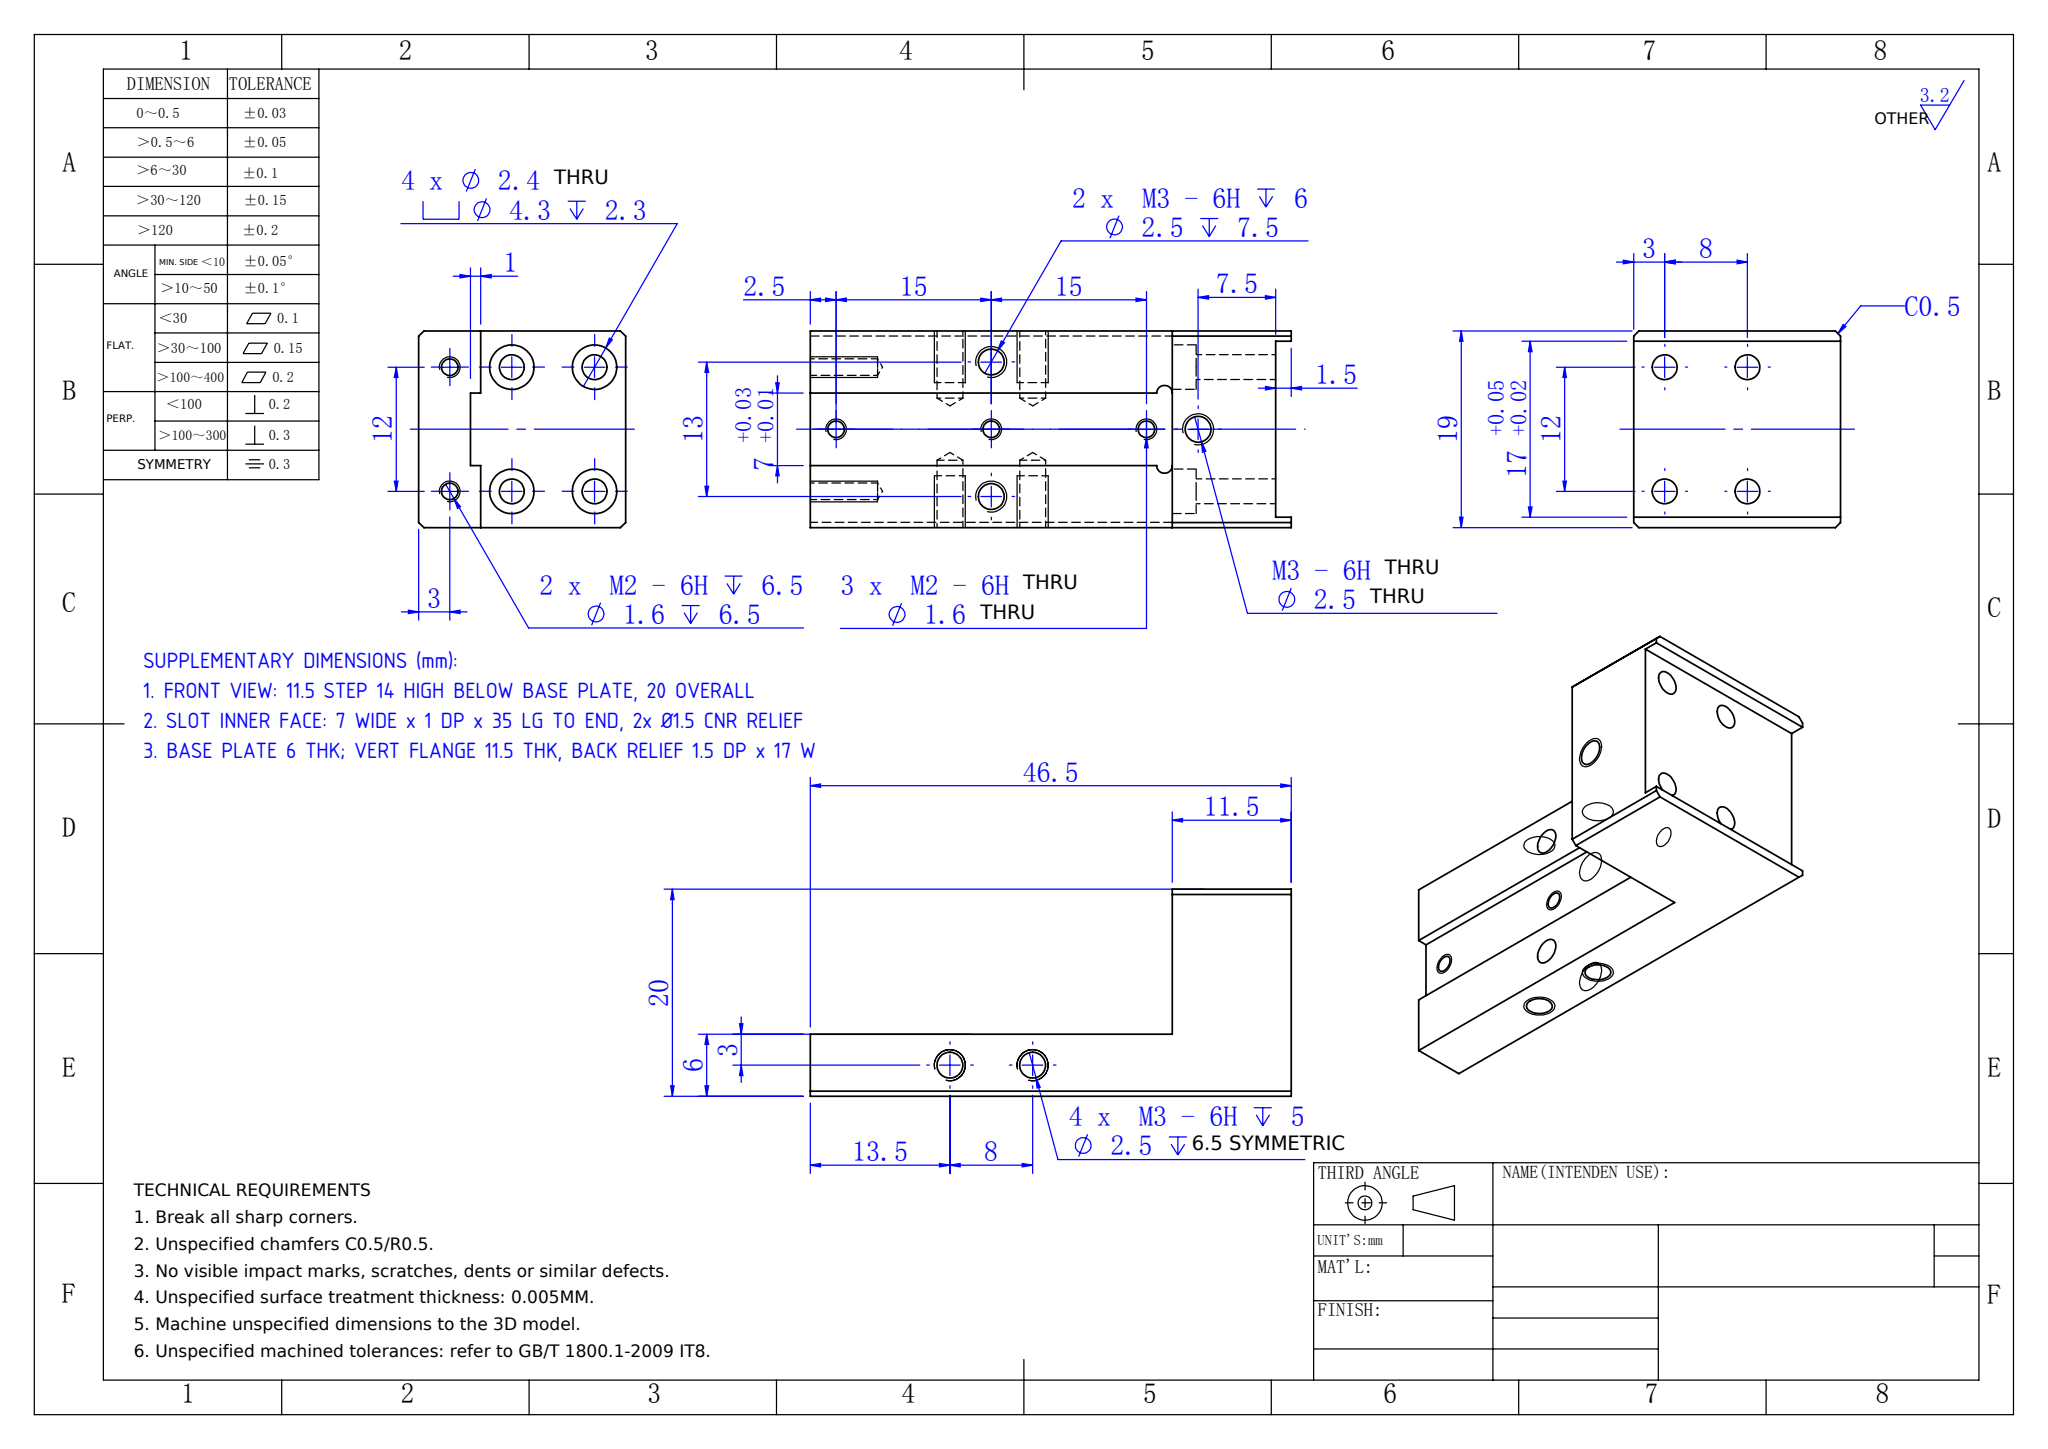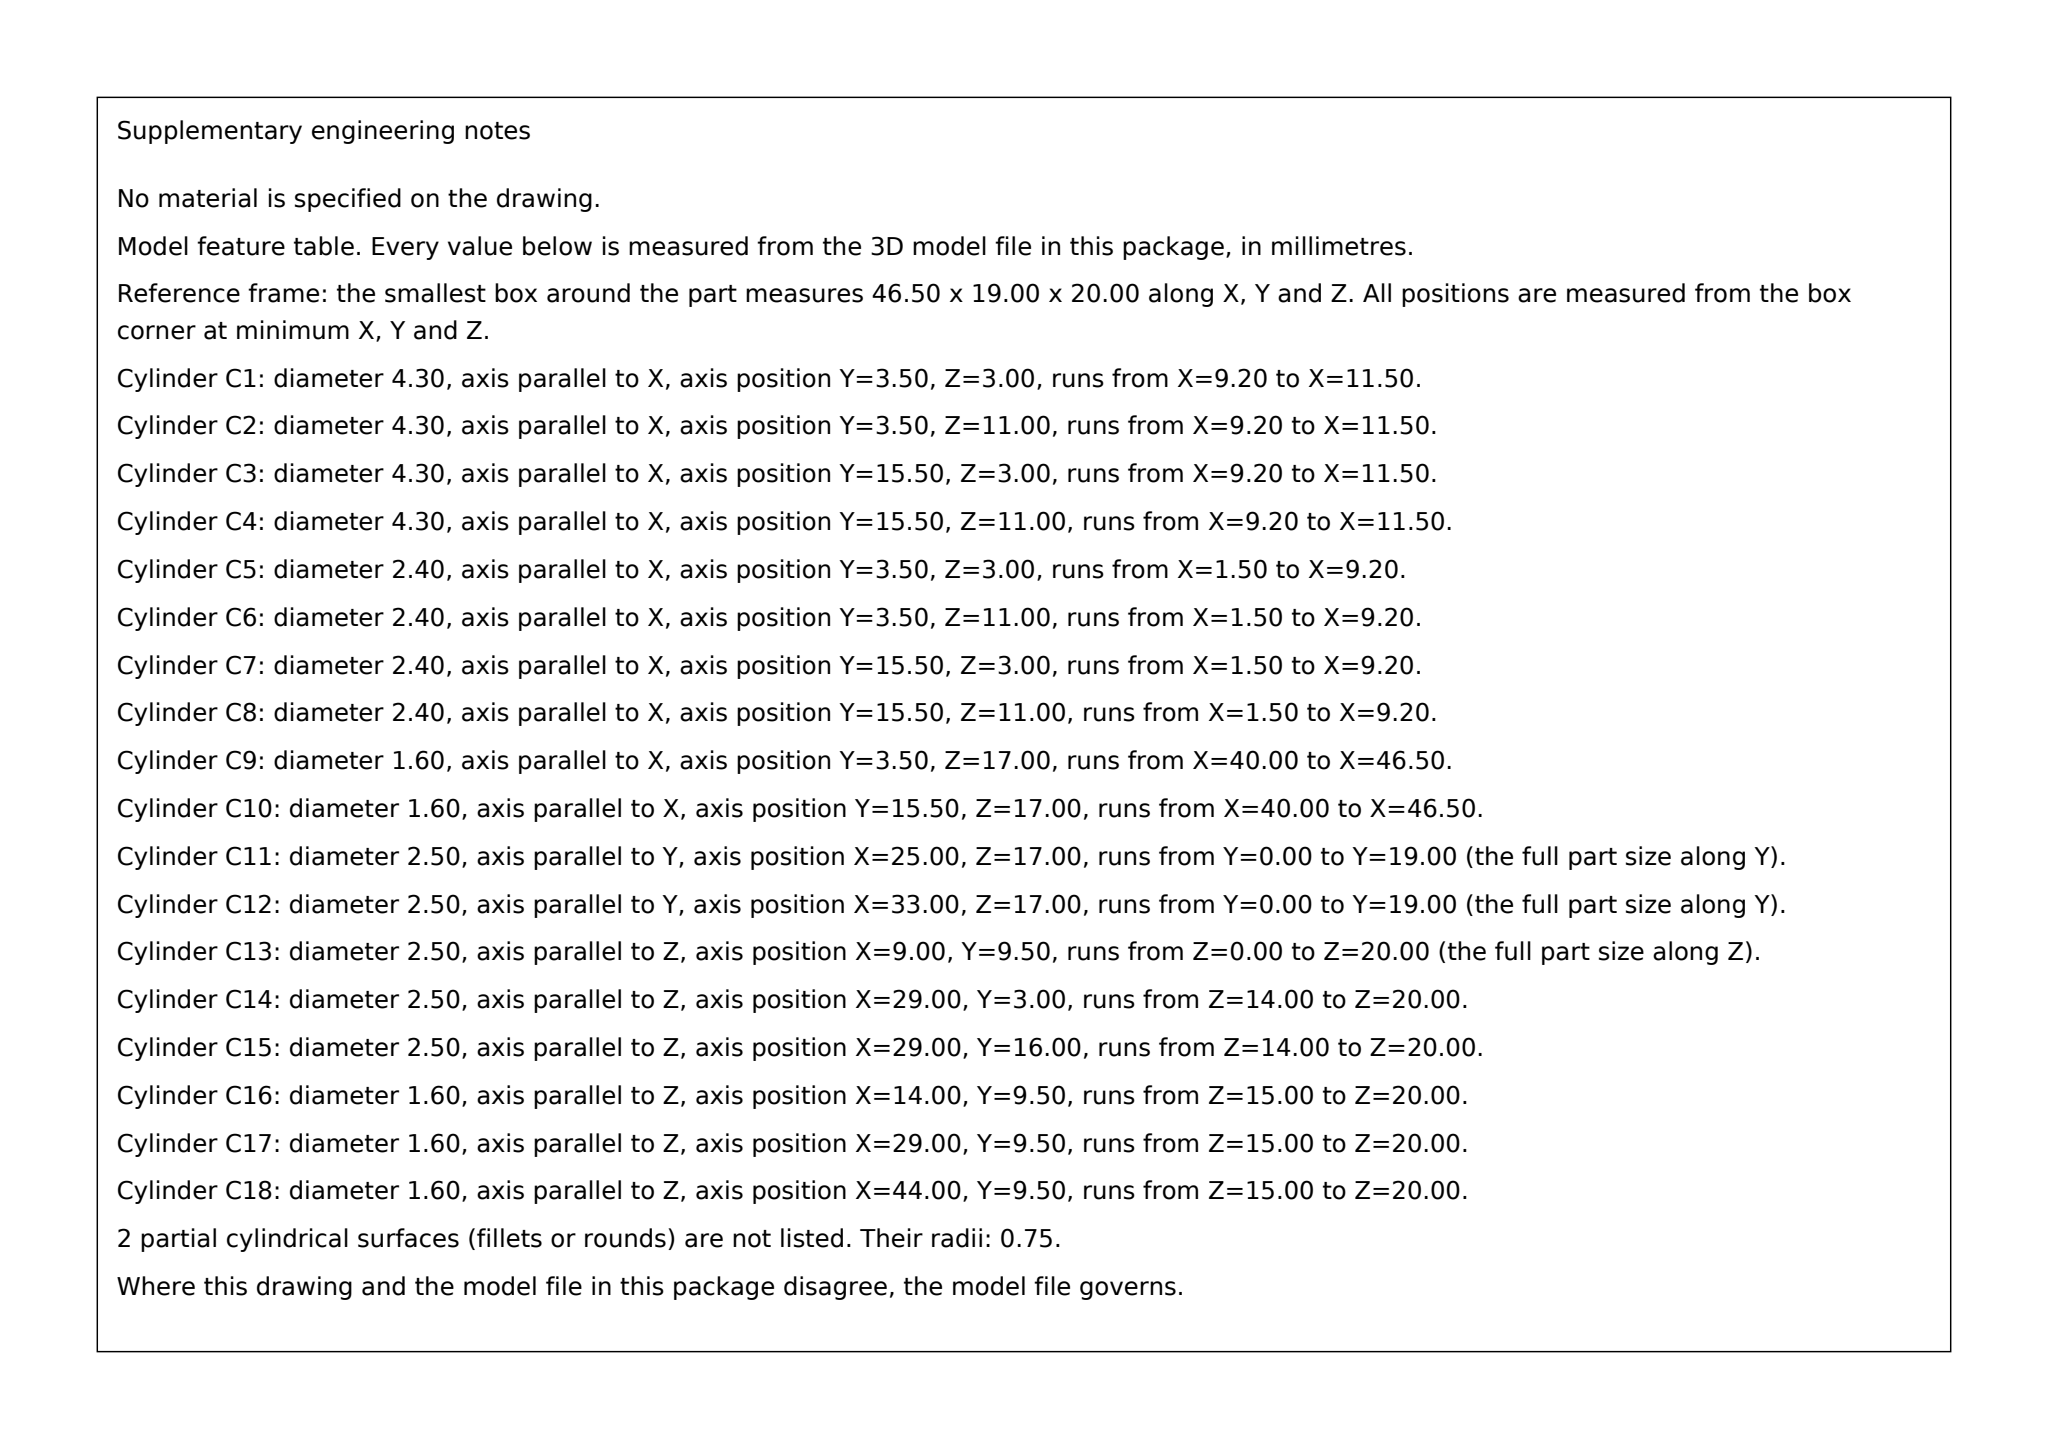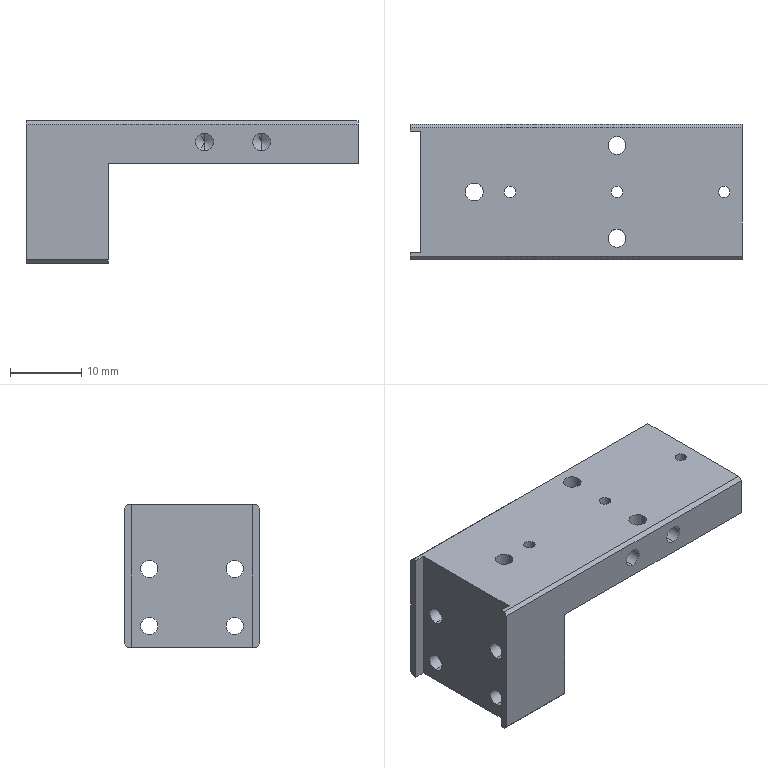Part | SolidWorks | mm | 1 solid | 78 faces | box 46.5 x 19 x 20 mm | volume 6969 mm3 | cylinder 42 | plane 24 | cone 12 | commonest cylinder face diameters 2.5 x14 1.6 x10 4.3 x8 2.4 x8 1.5 x2
build123d program:
from build123d import *

# Parameters (mm, degrees)
SKETCH1_W                                            = 35
SKETCH1_H                                            = 19
BOSS_EXTRUDE1_DEPTH                                  = 4
SKETCH3_W                                            = 4.5
SKETCH3_H                                            = 19
BOSS_EXTRUDE2_DEPTH                                  = 16
CUT_EXTRUDE1_DEPTH                                   = 1
M3_CLEARANCE_HOLE_1_D                                = 3.4
SKETCH9_W                                            = 39.5
SKETCH9_H                                            = 19
BOSS_EXTRUDE3_DEPTH                                  = 2
M2_TAPPED_HOLE2_D                                    = 1.6
SKETCH19_W                                           = 20
SKETCH19_H                                           = 19
BOSS_EXTRUDE4_DEPTH                                  = 10
HOLE_SIZE_ACCORDING_TO_THE_TYPE_OF_HEXAG_D           = 2.4
HOLE_SIZE_ACCORDING_TO_THE_TYPE_OF_HEXAG_DEPTH       = 10
HOLE_SIZE_ACCORDING_TO_THE_TYPE_OF_HEXAG_CBORE_D     = 4.3
HOLE_SIZE_ACCORDING_TO_THE_TYPE_OF_HEXAG_CBORE_DEPTH = 2.3
SKETCH22_W                                           = 20
SKETCH22_H                                           = 1
BOSS_EXTRUDE5_DEPTH                                  = 1.5
M3_TAPPED_HOLE2_D                                    = 2.5
M3_TAPPED_HOLE2_DEPTH                                = 7.5
M3_TAPPED_HOLE2_TIP                                  = 0.7511
CHAMFER1_SIZE                                        = 0.5
M3_TAPPED_HOLE3_D                                    = 2.5
SKETCH30_W                                           = 13.082
SKETCH30_H                                           = 35.173
CUT_EXTRUDE2_DEPTH                                   = 36.43
M2_TAPPED_HOLE4_D                                    = 1.6
M2_TAPPED_HOLE4_DEPTH                                = 6.5
M2_TAPPED_HOLE4_TIP                                  = 0.4807
M3_TAPPED_HOLE4_AT_2_COUNT                           = 2
M3_TAPPED_HOLE4_AT_2_PITCH                           = 8


with BuildPart() as part:
    # Sketch1 → Boss-Extrude1 (new body)
    with BuildSketch(Plane.XY):
        Rectangle(SKETCH1_W, SKETCH1_H)
    extrude(amount=BOSS_EXTRUDE1_DEPTH)

    # Sketch3 → Boss-Extrude2 (add)
    with BuildSketch(Plane.XY.offset(4)):
        with Locations((19.75, 0)):
            Rectangle(SKETCH3_W, SKETCH3_H)
    extrude(amount=-BOSS_EXTRUDE2_DEPTH)

    # Sketch4 → Cut-Extrude1 (cut)
    with BuildSketch(Plane(origin=(0, 0, 0), x_dir=(-1, 0, 0), z_dir=(0, 0, -1))):
        with BuildLine():
            Line((16, -3.5), (-17.5, -3.5))
            Line((-17.5, -3.5), (-17.5, 3.5))
            Line((-17.5, 3.5), (16, 3.5))
            ThreePointArc((16, 3.5), (16.75, 4.25), (17.5, 3.5))
            Line((17.5, 3.5), (17.5, -3.5))
            ThreePointArc((17.5, -3.5), (16.75, -4.25), (16, -3.5))
        make_face()
    extrude(amount=-CUT_EXTRUDE1_DEPTH, mode=Mode.SUBTRACT)

    # M3 Clearance Hole 1 (through all)
    with Locations(Plane(origin=(22, 0, 0), x_dir=(0, 0, -1), z_dir=(1, 0, 0))):
        with Locations((9.5, 0)):
            Hole(M3_CLEARANCE_HOLE_1_D / 2)

    # Sketch9 → Boss-Extrude3 (add)
    with BuildSketch(Plane.XY.offset(4)):
        with Locations((2.25, 0)):
            Rectangle(SKETCH9_W, SKETCH9_H)
    extrude(amount=BOSS_EXTRUDE3_DEPTH)

    # M2 Tapped Hole2 (through all)
    with Locations(Plane(origin=(0, 0, 0), x_dir=(-1, 0, 0), z_dir=(0, 0, -1))):
        with Locations((0, 0), (15, 0), (-15, 0)):
            Hole(M2_TAPPED_HOLE2_D / 2)

    # Sketch19 → Boss-Extrude4 (add)
    with BuildSketch(Plane.ZY.offset(17.5)):
        with Locations((-4, 0)):
            Rectangle(SKETCH19_W, SKETCH19_H)
    extrude(amount=BOSS_EXTRUDE4_DEPTH)

    # Hole Size according to the type of hexag
    with Locations(Plane(origin=(-17.5, 0, 0), x_dir=(0, 0, -1), z_dir=(1, 0, 0))):
        with Locations((11, -6), (3, -6), (3, 6), (11, 6)):
            CounterBoreHole(HOLE_SIZE_ACCORDING_TO_THE_TYPE_OF_HEXAG_D / 2, HOLE_SIZE_ACCORDING_TO_THE_TYPE_OF_HEXAG_CBORE_D / 2, HOLE_SIZE_ACCORDING_TO_THE_TYPE_OF_HEXAG_CBORE_DEPTH, depth=HOLE_SIZE_ACCORDING_TO_THE_TYPE_OF_HEXAG_DEPTH)

    # Sketch22 → Boss-Extrude5 (add)
    with BuildSketch(Plane.ZY.offset(27.5)):
        with Locations((-4, -9)):
            Rectangle(SKETCH22_W, SKETCH22_H)
        with Locations((-4, 9)):
            Rectangle(SKETCH22_W, SKETCH22_H)
    extrude(amount=BOSS_EXTRUDE5_DEPTH)

    # M3 Tapped Hole2
    with Locations(Plane.XY.offset(6)):
        with Locations((0, -6.5), (0, 6.5)):
            Hole(M3_TAPPED_HOLE2_D / 2, depth=M3_TAPPED_HOLE2_DEPTH)
            with Locations((0, 0, -(M3_TAPPED_HOLE2_DEPTH + M3_TAPPED_HOLE2_TIP / 2))):  # 118° drill point
                Cone(0, M3_TAPPED_HOLE2_D / 2, M3_TAPPED_HOLE2_TIP, mode=Mode.SUBTRACT)

    # Chamfer1
    chamfer1_edges = [part.edges().sort_by_distance(p)[0] for p in [
        (-3.5, 9.5, 6),
        (-3.5, -9.5, 6),
        (-23.25, -9.5, -14),
        (-23.25, 9.5, -14),
        (19.75, -9.5, -12),
        (19.75, 9.5, -12),
    ]]
    chamfer(chamfer1_edges, length=CHAMFER1_SIZE)

    # M3 Tapped Hole3 (through all)
    with Locations(Plane(origin=(0, 0, -14), x_dir=(-1, 0, 0), z_dir=(0, 0, -1))):
        with Locations((20, 0)):
            Hole(M3_TAPPED_HOLE3_D / 2)

    # Sketch30 → Cut-Extrude2 (cut, through all)
    with BuildSketch(Plane(origin=(0, 0, -12), x_dir=(-1, 0, 0), z_dir=(0, 0, -1))):
        with Locations((-24.041, 4.281)):
            Rectangle(SKETCH30_W, SKETCH30_H)
    extrude(amount=-CUT_EXTRUDE2_DEPTH, mode=Mode.SUBTRACT)

    # M2 Tapped Hole4
    with Locations(Plane(origin=(17.5, 0, 0), x_dir=(0, 0, -1), z_dir=(1, 0, 0))):
        with Locations((-3, 6), (-3, -6)):
            Hole(M2_TAPPED_HOLE4_D / 2, depth=M2_TAPPED_HOLE4_DEPTH)
            with Locations((0, 0, -(M2_TAPPED_HOLE4_DEPTH + M2_TAPPED_HOLE4_TIP / 2))):  # 118° drill point
                Cone(0, M2_TAPPED_HOLE4_D / 2, M2_TAPPED_HOLE4_TIP, mode=Mode.SUBTRACT)

    # Sketch33 → M3 Tapped Hole4 (revolve, cut)
    with BuildSketch(Plane(origin=(4, 9.5, 3), x_dir=(0, 0, 1), z_dir=(1, 0, 0))):
        Polygon((0, 0), (0, 7.251), (1.25, 6.5), (1.25, 0), align=None)
    m3_tapped_hole4 = revolve(axis=Axis((4, 15.85, 3), (0, -1, 0)), mode=Mode.SUBTRACT)

    # M3 Tapped Hole4 at 2: M3 Tapped Hole4 ×2
    with Locations(*[(-i * M3_TAPPED_HOLE4_AT_2_PITCH, 0, 0) for i in range(1, M3_TAPPED_HOLE4_AT_2_COUNT)]):
        add(m3_tapped_hole4, mode=Mode.SUBTRACT)

    # Mirror1: M3 Tapped Hole4 across plane
    add(m3_tapped_hole4.mirror(Plane(origin=(0, 0, 0), x_dir=(0, 0, 1), z_dir=(0, -1, 0))), mode=Mode.SUBTRACT)

    # Mirror1 copy 1 sketch → Mirror1 copy 1 (revolve, cut)
    with BuildSketch(Plane(origin=(-4, -9.5, 3), x_dir=(0, 0, 1), z_dir=(1, 0, 0))):
        Polygon((0, 0), (0, -7.251), (1.25, -6.5), (1.25, 0), align=None)
    revolve(axis=Axis((-4, -15.85, 3), (0, -1, 0)), mode=Mode.SUBTRACT)


solid = part.part